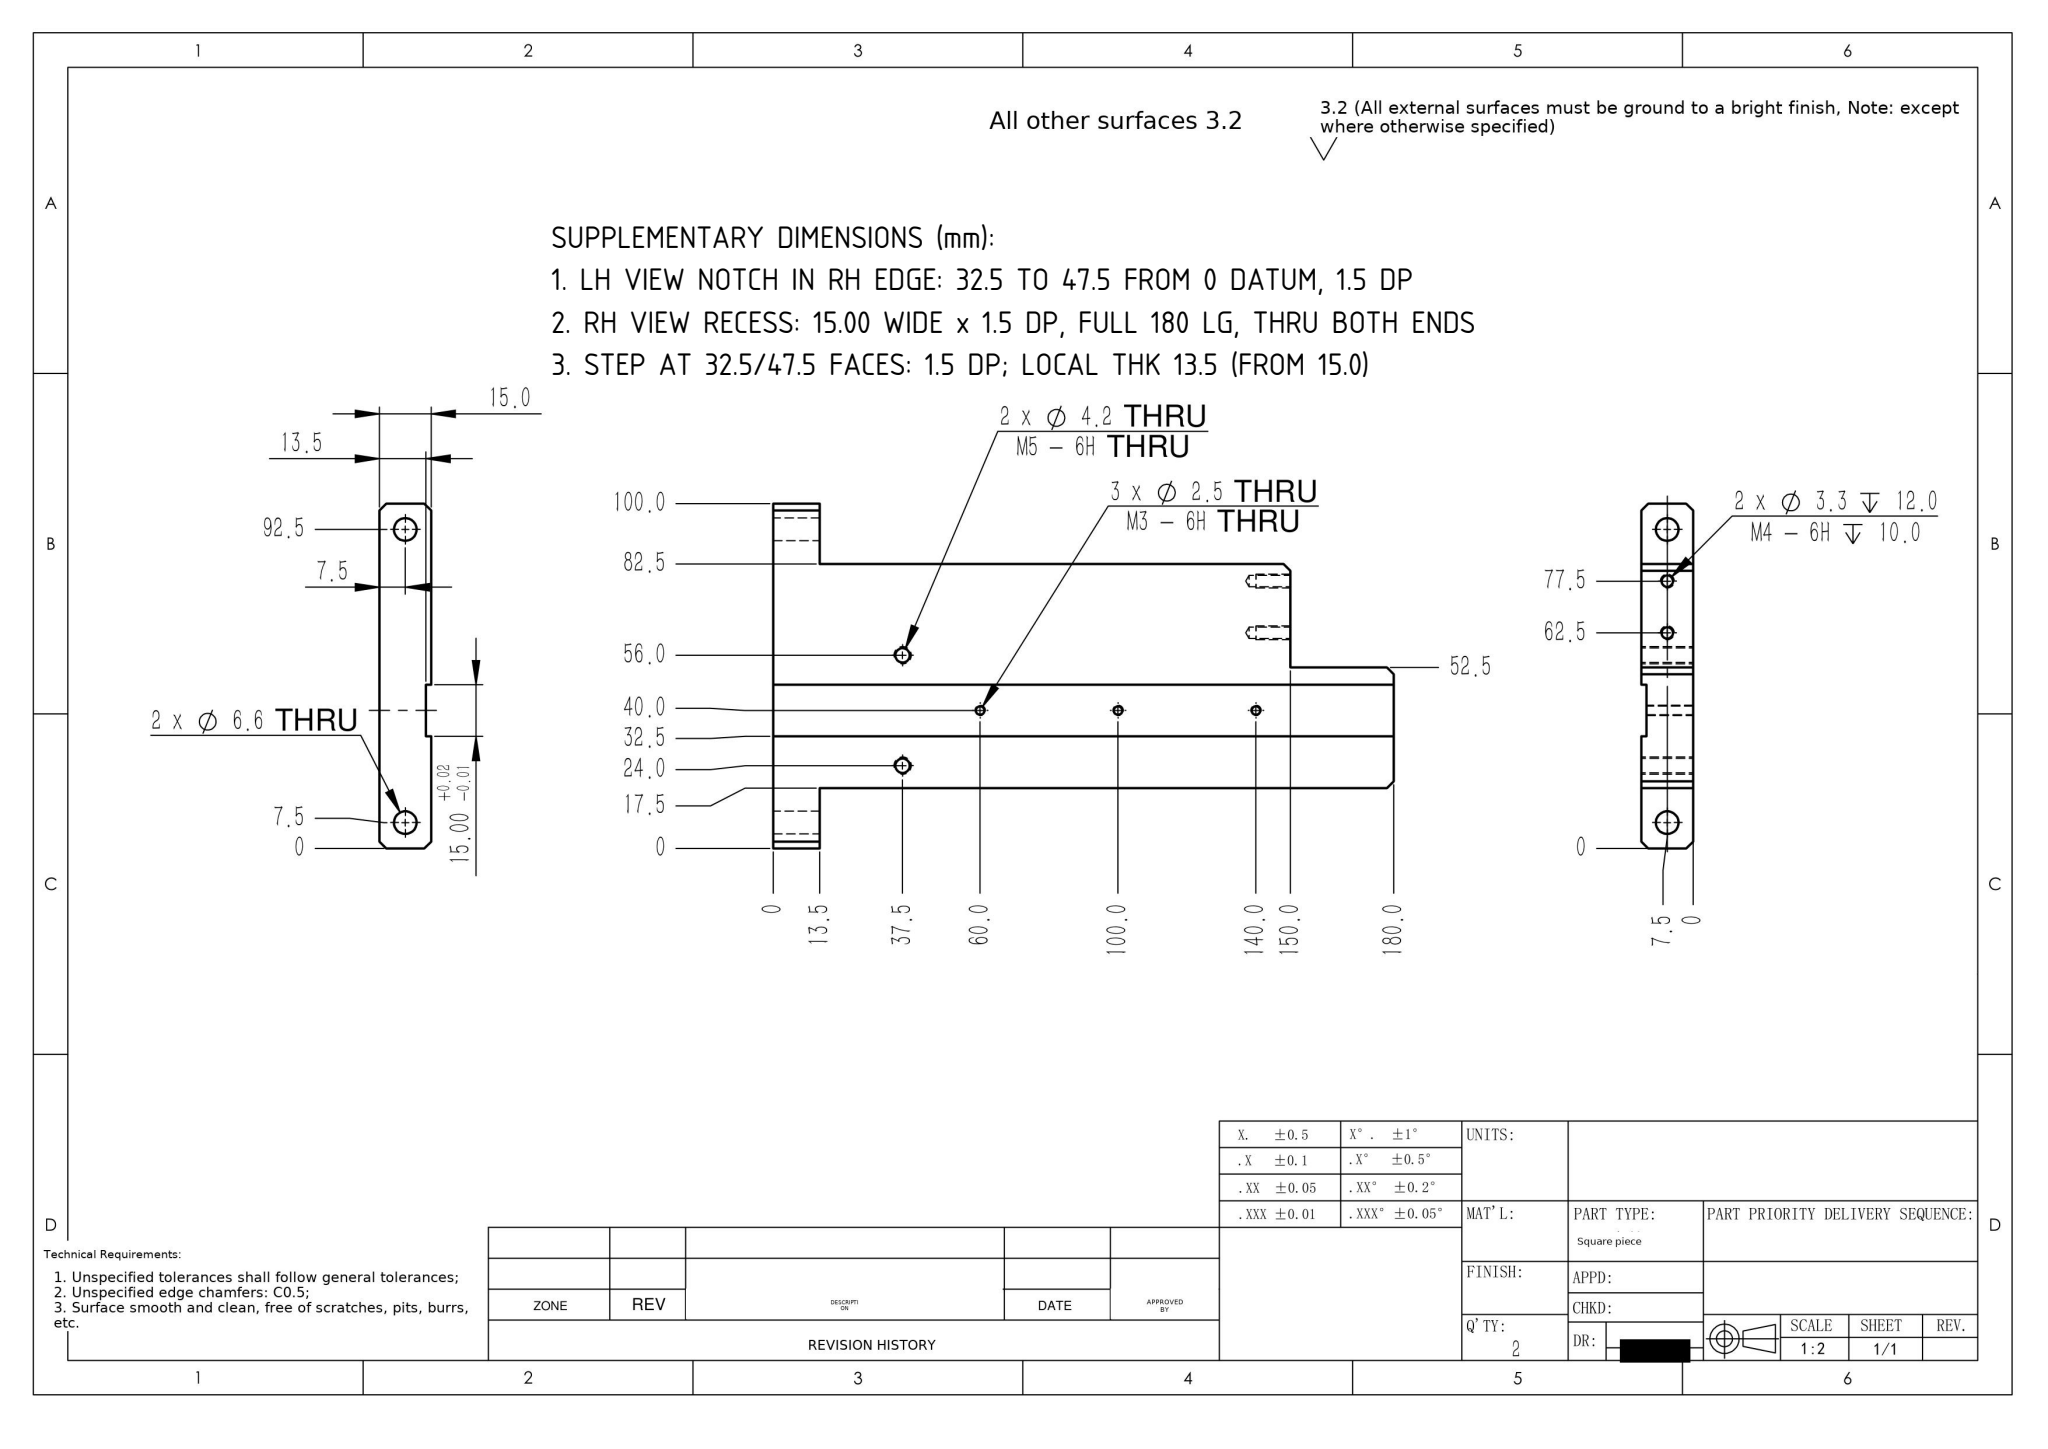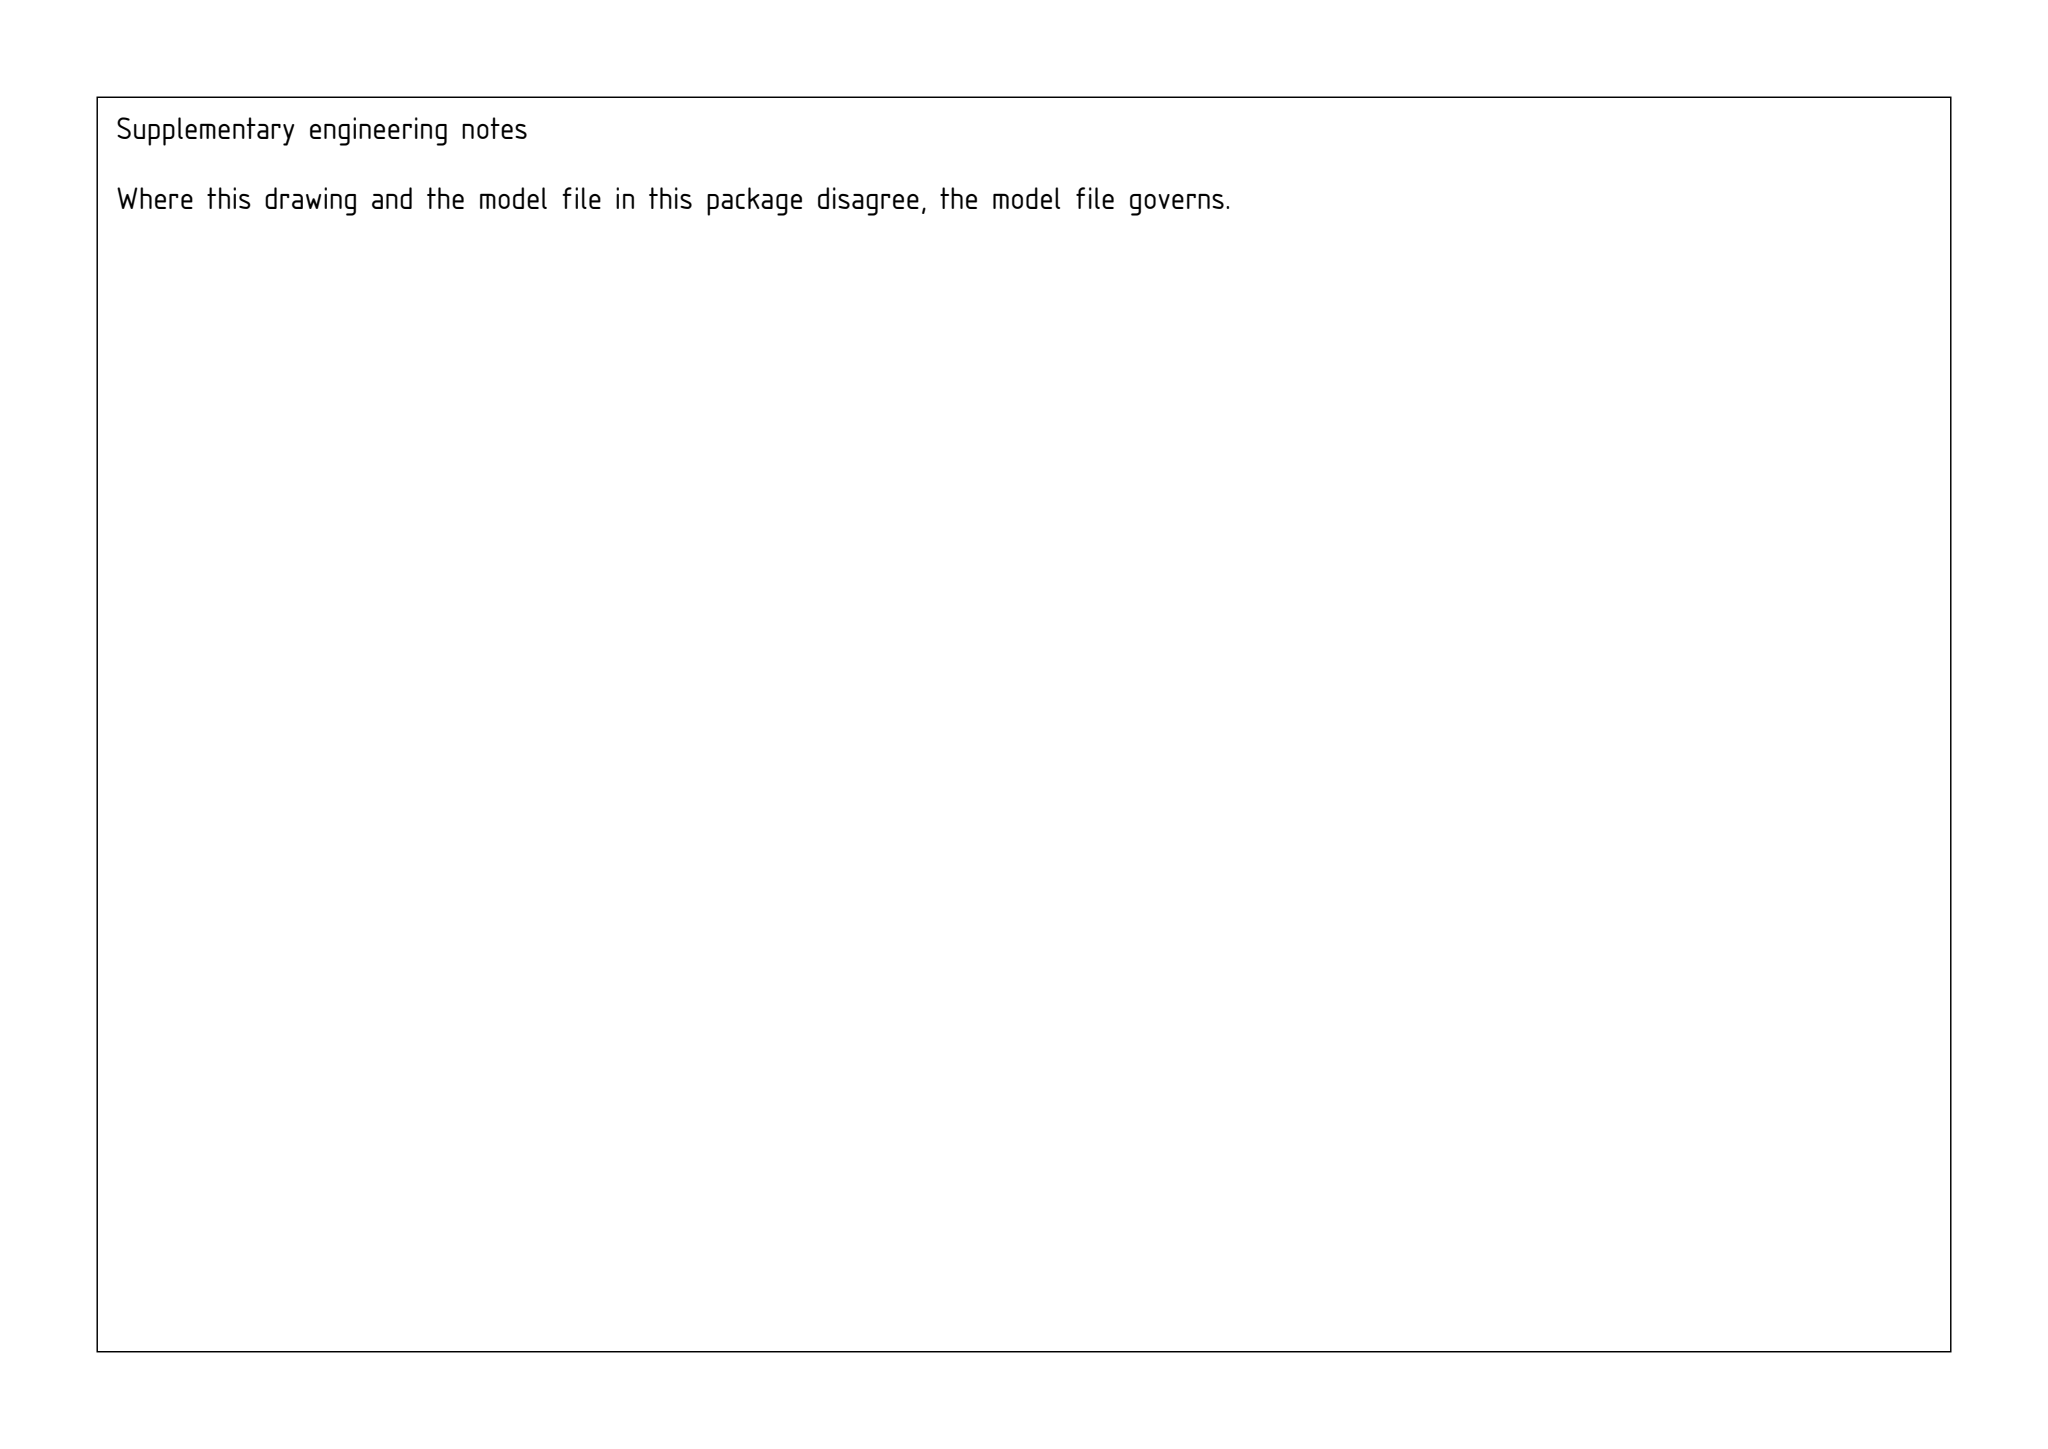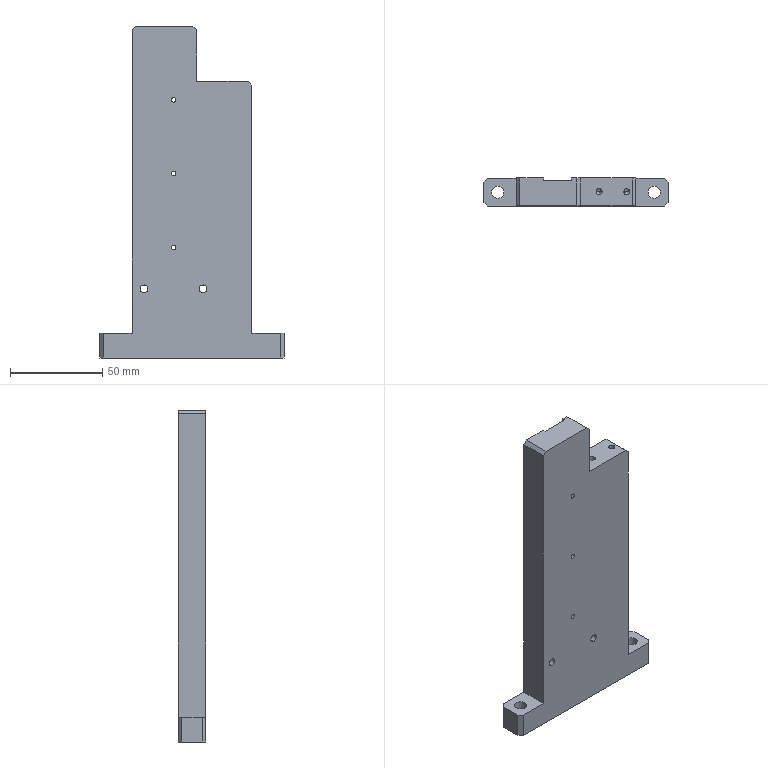Part | SolidWorks | mm | 1 solid | 45 faces | box 100 x 15 x 180 mm | volume 163090 mm3 | plane 23 | cylinder 18 | cone 4 | commonest cylinder face diameters 2.5 x6 4.2 x4 3.3 x4 6.6 x4
build123d program:
from build123d import *

# Parameters (mm, degrees)
SKETCH1_W             = 100
SKETCH1_H             = 15
BOSS_EXTRUDE1_DEPTH   = 180
SKETCH2_W             = 17.5
SKETCH2_H             = 166.5
CUT_EXTRUDE1_DEPTH    = 188.417
SKETCH11_W            = 30
SKETCH11_H            = 30
CUT_EXTRUDE3_DEPTH    = 188.417
M6_CLEARANCE_HOLE1_D  = 6.6
SKETCH6_W             = 15
SKETCH6_H             = 180
CUT_EXTRUDE2_DEPTH    = 1.5
M3_TAPPED_HOLE1_D     = 2.5
M4_TAPPED_HOLE1_D     = 3.3
M4_TAPPED_HOLE1_DEPTH = 12
M4_TAPPED_HOLE1_TIP   = 0.9914
M5_TAPPED_HOLE1_D     = 4.2
CHAMFER1_SIZE         = 2


with BuildPart() as part:
    # Sketch1 → Boss-Extrude1 (new body)
    with BuildSketch(Plane.XY):
        Rectangle(SKETCH1_W, SKETCH1_H)
    extrude(amount=BOSS_EXTRUDE1_DEPTH)

    # Sketch2 → Cut-Extrude1 (cut, through all)
    with BuildSketch(Plane(origin=(0, 7.5, 0), x_dir=(1, 0, 0), z_dir=(0, 1, 0))):
        with Locations((41.25, -96.75)):
            Rectangle(SKETCH2_W, SKETCH2_H)
        with Locations((-41.25, -96.75)):
            Rectangle(SKETCH2_W, SKETCH2_H)
    extrude(amount=-CUT_EXTRUDE1_DEPTH, mode=Mode.SUBTRACT)

    # Sketch11 → Cut-Extrude3 (cut, through all)
    with BuildSketch(Plane(origin=(0, 7.5, 0), x_dir=(1, 0, 0), z_dir=(0, 1, 0))):
        with Locations((17.5, -165)):
            Rectangle(SKETCH11_W, SKETCH11_H)
    extrude(amount=-CUT_EXTRUDE3_DEPTH, mode=Mode.SUBTRACT)

    # M6 Clearance Hole1 (through all)
    with Locations(Plane(origin=(0, 0, 0), x_dir=(-1, 0, 0), z_dir=(0, 0, -1))):
        with Locations((-42.5, 0), (42.5, 0)):
            Hole(M6_CLEARANCE_HOLE1_D / 2)

    # Sketch6 → Cut-Extrude2 (cut)
    with BuildSketch(Plane(origin=(0, 7.5, 0), x_dir=(1, 0, 0), z_dir=(0, 1, 0))):
        with Locations((-10, -90)):
            Rectangle(SKETCH6_W, SKETCH6_H)
    extrude(amount=-CUT_EXTRUDE2_DEPTH, mode=Mode.SUBTRACT)

    # M3 Tapped Hole1 (through all)
    with Locations(Plane(origin=(0, 7.5, 0), x_dir=(1, 0, 0), z_dir=(0, 1, 0))):
        with Locations((-10, -60), (-10, -100), (-10, -140)):
            Hole(M3_TAPPED_HOLE1_D / 2)

    # M4 Tapped Hole1
    with Locations(Plane.XY.offset(150)):
        with Locations((12.5, 0), (27.5, 0)):
            Hole(M4_TAPPED_HOLE1_D / 2, depth=M4_TAPPED_HOLE1_DEPTH)
            with Locations((0, 0, -(M4_TAPPED_HOLE1_DEPTH + M4_TAPPED_HOLE1_TIP / 2))):  # 118° drill point
                Cone(0, M4_TAPPED_HOLE1_D / 2, M4_TAPPED_HOLE1_TIP, mode=Mode.SUBTRACT)

    # M5 Tapped Hole1 (through all)
    with Locations(Plane(origin=(0, 7.5, 0), x_dir=(1, 0, 0), z_dir=(0, 1, 0))):
        with Locations((6, -37.5), (-26, -37.5)):
            Hole(M5_TAPPED_HOLE1_D / 2)

    # Chamfer1
    chamfer1_edges = [part.edges().sort_by_distance(p)[0] for p in [
        (50, -7.5, 6.75),
        (50, 7.5, 6.75),
        (-50, -7.5, 6.75),
        (-50, 7.5, 6.75),
        (-32.5, 0, 180),
        (32.5, 0, 150),
        (2.5, 0, 180),
    ]]
    chamfer(chamfer1_edges, length=CHAMFER1_SIZE)


solid = part.part